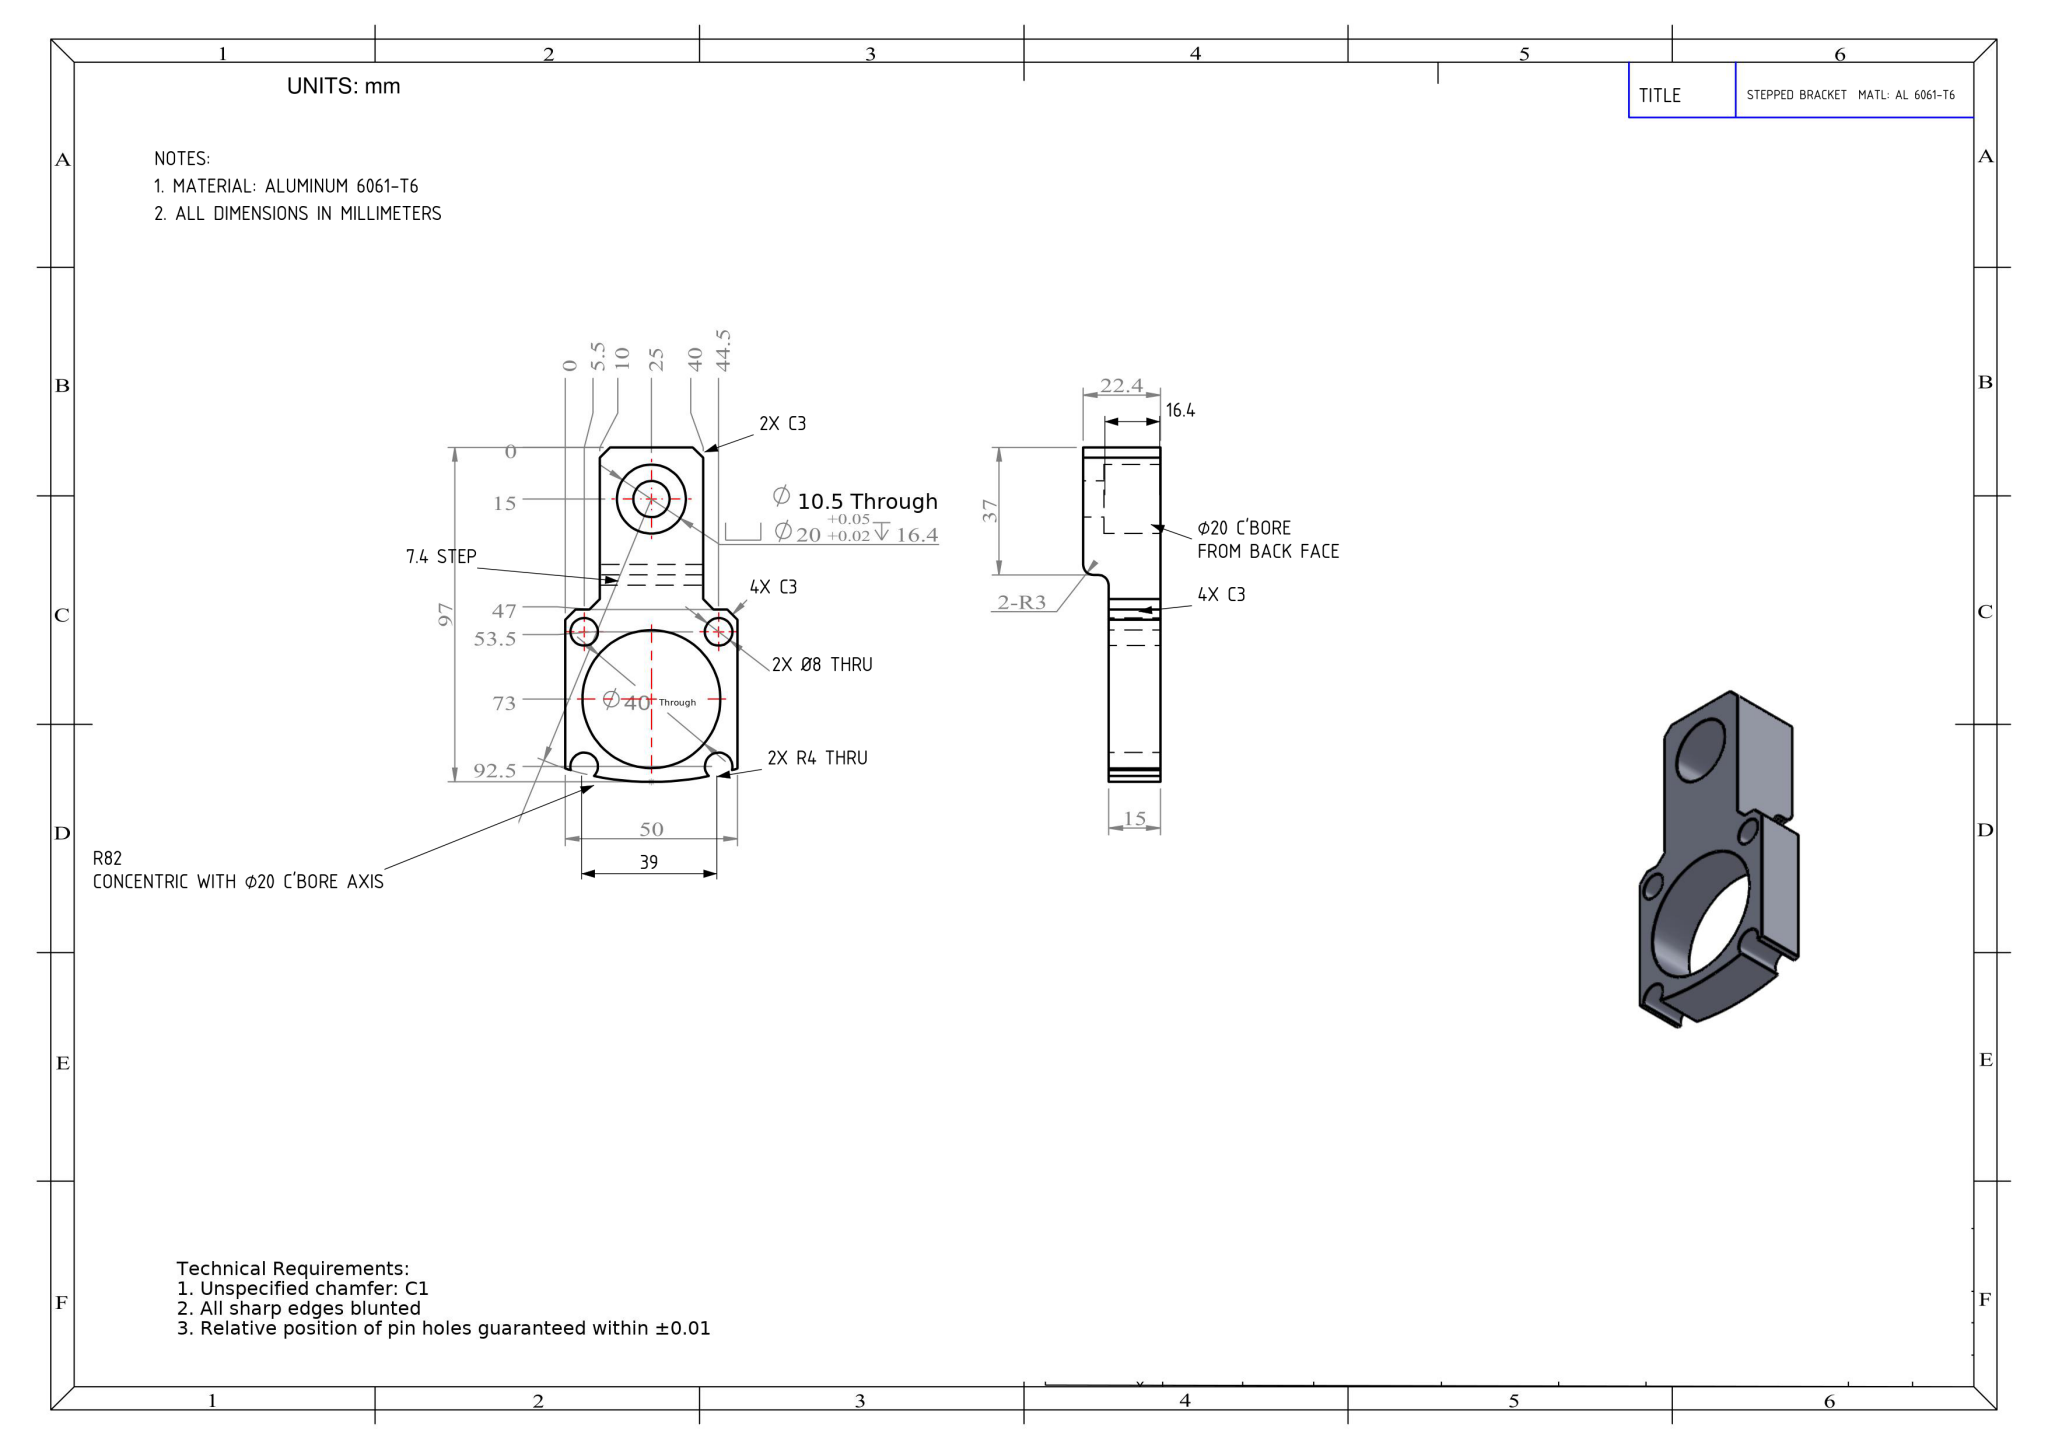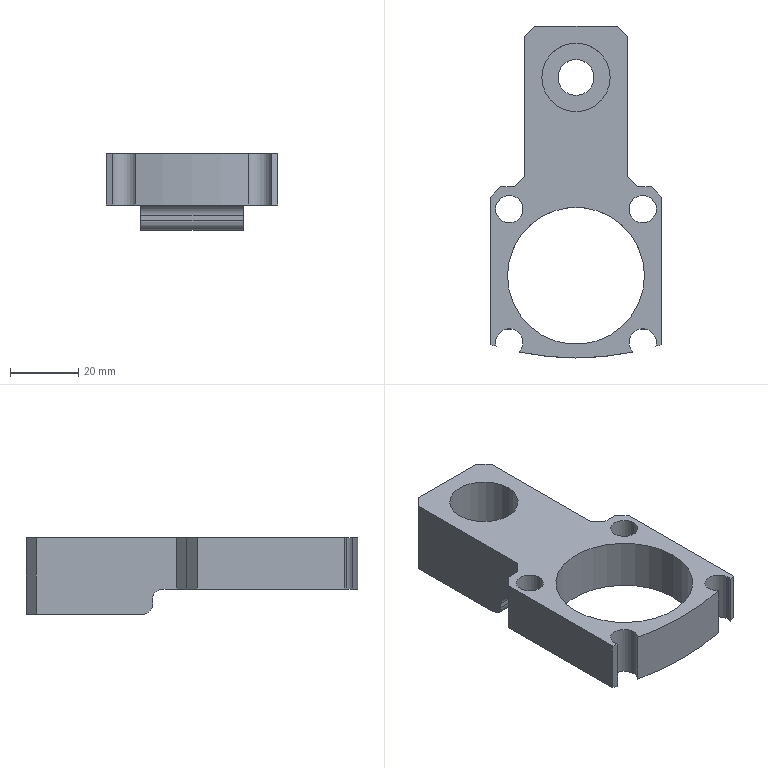Part | NX | mm | 1 solid | 39 faces | box 50 x 97 x 22.4 mm | volume 38441 mm3 | cylinder 21 | plane 18 | commonest cylinder face diameters 8 x10 164 x3 40 x2 10.5 x2 20 x2 6 x2